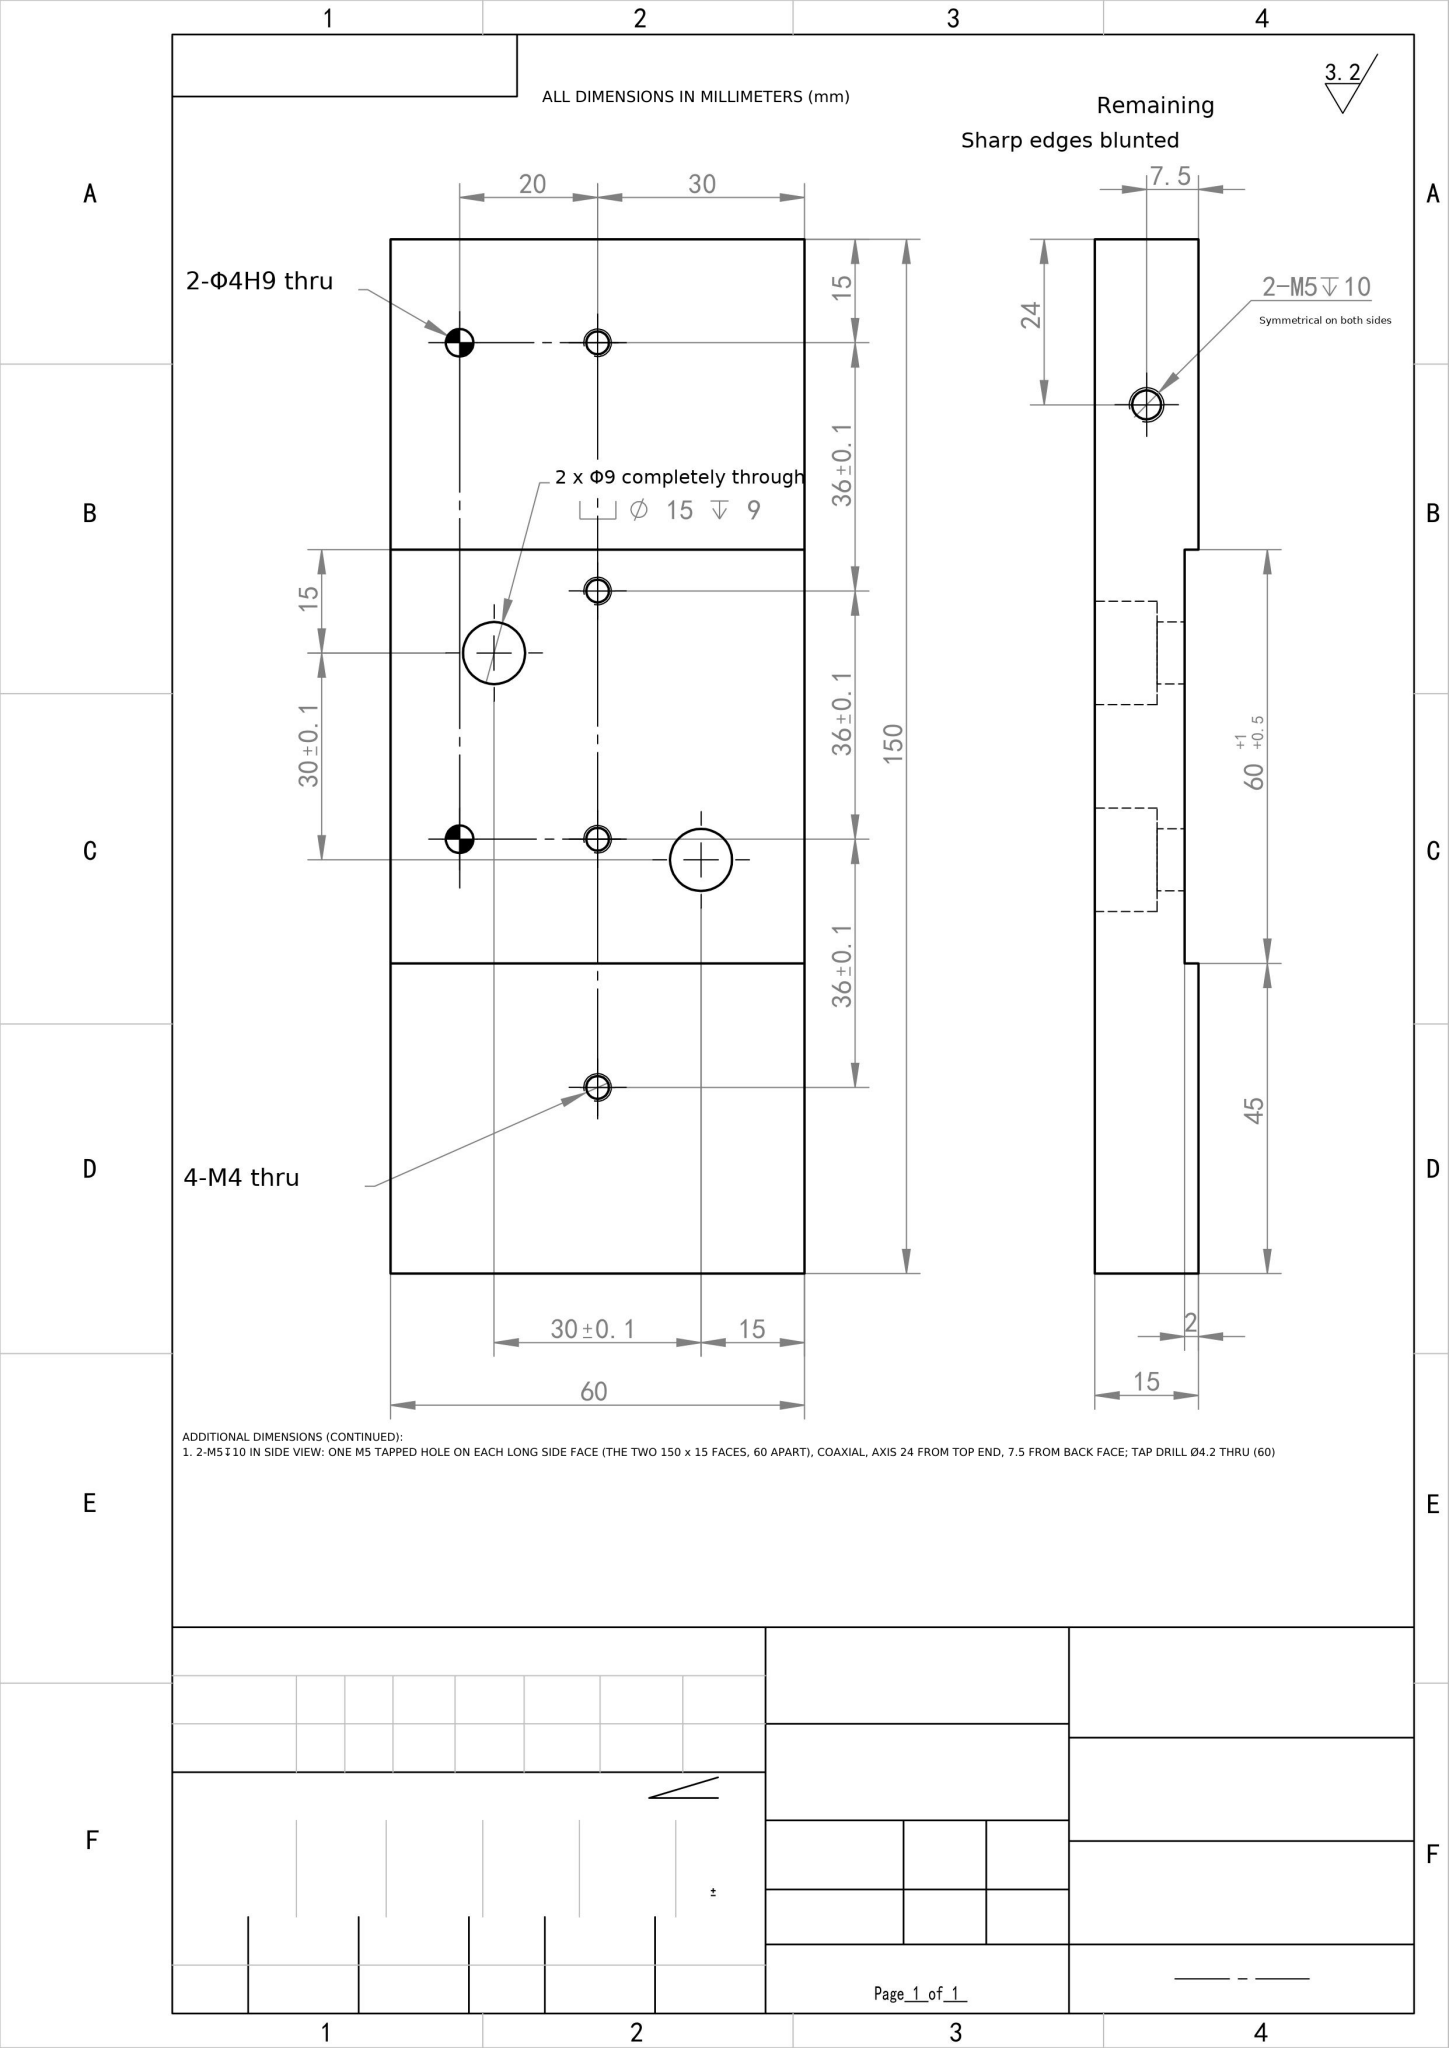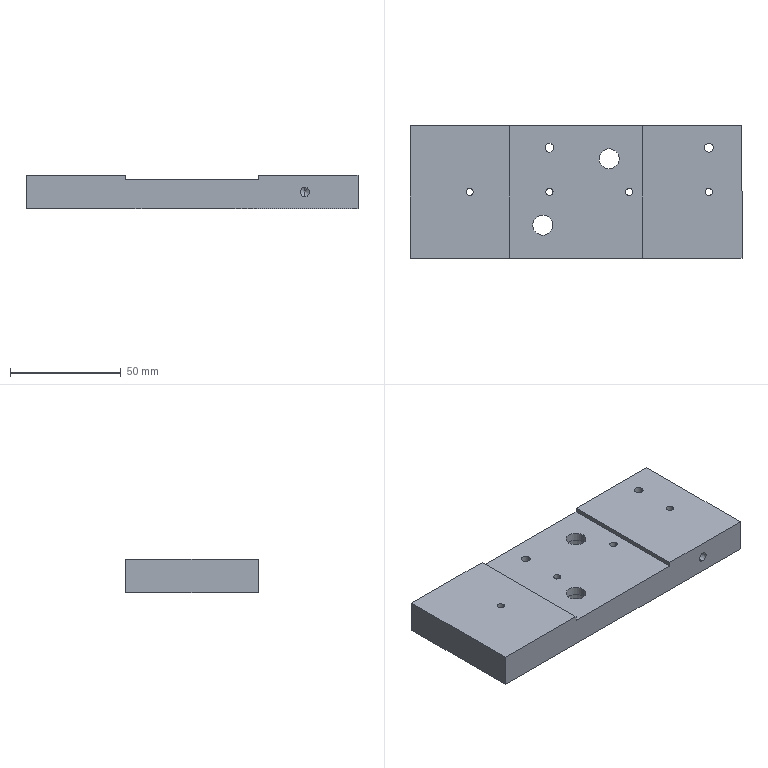Part | NX | mm | 1 solid | 40 faces | box 150 x 60 x 15 mm | volume 122880 mm3 | cylinder 24 | plane 12 | cone 4 | commonest cylinder face diameters 3.3 x8 4.2 x4 15 x4 9 x4 4 x4